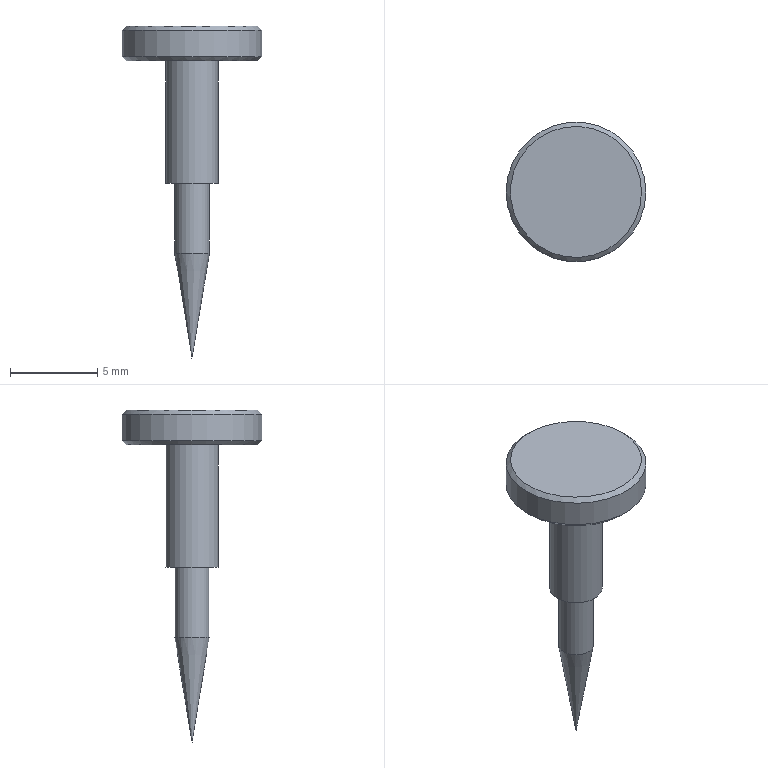Component | NX | AIR_PUMP_PART_01_20 | 1 solid | 9 faces | box 8 x 8 x 19 mm | volume 167 mm3 | cone 3 | cylinder 3 | plane 3 | commonest cylinder face diameters 2 x1 3 x1 8 x1
STEP:
#1=CARTESIAN_POINT('',(0.,0.,0.));
#2=DIRECTION('',(0.,0.,1.));
#3=DIRECTION('',(1.,0.,0.));
#4=AXIS2_PLACEMENT_3D('',#1,#2,#3);
#5=CARTESIAN_POINT('',(0.0005589,-32.2,83.052));
#6=VERTEX_POINT('',#5);
#7=CARTESIAN_POINT('',(1.001,-32.2,89.052));
#8=VERTEX_POINT('',#7);
#9=CARTESIAN_POINT('',(0.0005589,-32.2,83.052));
#10=CARTESIAN_POINT('',(1.001,-32.2,89.052));
#11=B_SPLINE_CURVE_WITH_KNOTS('',1,(#9,#10),.UNSPECIFIED.,.F.,.F.,(2,2),(-6.083,0.),.PIECEWISE_BEZIER_KNOTS.);
#12=CARTESIAN_POINT('',(0.0005589,-32.2,89.052));
#13=DIRECTION('',(0.,0.,1.));
#14=DIRECTION('',(1.,0.,0.));
#15=AXIS2_PLACEMENT_3D('',#12,#13,#14);
#16=CONICAL_SURFACE('',#15,1.,0.1651);
#17=CARTESIAN_POINT('',(6.283,0.));
#18=DIRECTION('',(0.,1.));
#19=VECTOR('',#18,1.);
#20=LINE('',#17,#19);
#21=(GEOMETRIC_REPRESENTATION_CONTEXT(2)PARAMETRIC_REPRESENTATION_CONTEXT()REPRESENTATION_CONTEXT('',''));
#22=DEFINITIONAL_REPRESENTATION('',(#20),#21);
#23=PCURVE('',#16,#22);
#24=CARTESIAN_POINT('',(0.,0.));
#25=DIRECTION('',(0.,1.));
#26=VECTOR('',#25,1.);
#27=LINE('',#24,#26);
#28=(GEOMETRIC_REPRESENTATION_CONTEXT(2)PARAMETRIC_REPRESENTATION_CONTEXT()REPRESENTATION_CONTEXT('',''));
#29=DEFINITIONAL_REPRESENTATION('',(#27),#28);
#30=PCURVE('',#16,#29);
#31=SEAM_CURVE('',#11,(#23,#30),.PCURVE_S1.);
#32=EDGE_CURVE('',#6,#8,#31,.T.);
#33=ORIENTED_EDGE('',*,*,#32,.T.);
#34=CARTESIAN_POINT('',(0.0005589,-32.2,89.052));
#35=DIRECTION('',(0.,0.,1.));
#36=DIRECTION('',(1.,0.,0.));
#37=AXIS2_PLACEMENT_3D('',#34,#35,#36);
#38=CIRCLE('',#37,1.);
#39=CARTESIAN_POINT('',(0.,0.));
#40=DIRECTION('',(1.,0.));
#41=VECTOR('',#40,1.);
#42=LINE('',#39,#41);
#43=(GEOMETRIC_REPRESENTATION_CONTEXT(2)PARAMETRIC_REPRESENTATION_CONTEXT()REPRESENTATION_CONTEXT('',''));
#44=DEFINITIONAL_REPRESENTATION('',(#42),#43);
#45=PCURVE('',#16,#44);
#46=CARTESIAN_POINT('',(0.0005589,-32.2,83.052));
#47=DIRECTION('',(0.,0.,1.));
#48=DIRECTION('',(1.,0.,0.));
#49=AXIS2_PLACEMENT_3D('',#46,#47,#48);
#50=CYLINDRICAL_SURFACE('',#49,1.);
#51=CARTESIAN_POINT('',(0.,6.));
#52=DIRECTION('',(1.,0.));
#53=VECTOR('',#52,1.);
#54=LINE('',#51,#53);
#55=(GEOMETRIC_REPRESENTATION_CONTEXT(2)PARAMETRIC_REPRESENTATION_CONTEXT()REPRESENTATION_CONTEXT('',''));
#56=DEFINITIONAL_REPRESENTATION('',(#54),#55);
#57=PCURVE('',#50,#56);
#58=SURFACE_CURVE('',#38,(#45,#57),.PCURVE_S1.);
#59=EDGE_CURVE('',#8,#8,#58,.T.);
#60=ORIENTED_EDGE('',*,*,#59,.F.);
#61=ORIENTED_EDGE('',*,*,#32,.F.);
#62=EDGE_LOOP('',(#33,#60,#61));
#63=FACE_BOUND('',#62,.T.);
#64=ADVANCED_FACE('',(#63),#16,.T.);
#65=ORIENTED_EDGE('',*,*,#59,.T.);
#66=CARTESIAN_POINT('',(1.001,-32.2,93.052));
#67=VERTEX_POINT('',#66);
#68=CARTESIAN_POINT('',(1.001,-32.2,89.052));
#69=CARTESIAN_POINT('',(1.001,-32.2,93.052));
#70=B_SPLINE_CURVE_WITH_KNOTS('',1,(#68,#69),.UNSPECIFIED.,.F.,.F.,(2,2),(6.,10.),.PIECEWISE_BEZIER_KNOTS.);
#71=CARTESIAN_POINT('',(6.283,0.));
#72=DIRECTION('',(0.,1.));
#73=VECTOR('',#72,1.);
#74=LINE('',#71,#73);
#75=(GEOMETRIC_REPRESENTATION_CONTEXT(2)PARAMETRIC_REPRESENTATION_CONTEXT()REPRESENTATION_CONTEXT('',''));
#76=DEFINITIONAL_REPRESENTATION('',(#74),#75);
#77=PCURVE('',#50,#76);
#78=CARTESIAN_POINT('',(0.,0.));
#79=DIRECTION('',(0.,1.));
#80=VECTOR('',#79,1.);
#81=LINE('',#78,#80);
#82=(GEOMETRIC_REPRESENTATION_CONTEXT(2)PARAMETRIC_REPRESENTATION_CONTEXT()REPRESENTATION_CONTEXT('',''));
#83=DEFINITIONAL_REPRESENTATION('',(#81),#82);
#84=PCURVE('',#50,#83);
#85=SEAM_CURVE('',#70,(#77,#84),.PCURVE_S1.);
#86=EDGE_CURVE('',#8,#67,#85,.T.);
#87=ORIENTED_EDGE('',*,*,#86,.T.);
#88=CARTESIAN_POINT('',(0.0005589,-32.2,93.052));
#89=DIRECTION('',(0.,0.,1.));
#90=DIRECTION('',(1.,0.,0.));
#91=AXIS2_PLACEMENT_3D('',#88,#89,#90);
#92=CIRCLE('',#91,1.);
#93=CARTESIAN_POINT('',(0.,10.));
#94=DIRECTION('',(1.,0.));
#95=VECTOR('',#94,1.);
#96=LINE('',#93,#95);
#97=(GEOMETRIC_REPRESENTATION_CONTEXT(2)PARAMETRIC_REPRESENTATION_CONTEXT()REPRESENTATION_CONTEXT('',''));
#98=DEFINITIONAL_REPRESENTATION('',(#96),#97);
#99=PCURVE('',#50,#98);
#100=CARTESIAN_POINT('',(0.0005589,-33.7,93.052));
#101=DIRECTION('',(0.,0.,-1.));
#102=DIRECTION('',(-1.,0.,0.));
#103=AXIS2_PLACEMENT_3D('',#100,#101,#102);
#104=PLANE('',#103);
#105=CARTESIAN_POINT('',(-1.,1.5));
#106=CARTESIAN_POINT('',(-1.,3.232));
#107=CARTESIAN_POINT('',(0.5,2.366));
#108=CARTESIAN_POINT('',(2.,1.5));
#109=CARTESIAN_POINT('',(0.5,0.634));
#110=CARTESIAN_POINT('',(-1.,-0.2321));
#111=CARTESIAN_POINT('',(-1.,1.5));
#112=(BOUNDED_CURVE()B_SPLINE_CURVE(2,(#105,#106,#107,#108,#109,#110,#111),.UNSPECIFIED.,.T.,.F.)B_SPLINE_CURVE_WITH_KNOTS((1,2,2,2,2,1),(-2.094,0.,2.094,4.189,6.283,8.378),.UNSPECIFIED.)CURVE()GEOMETRIC_REPRESENTATION_ITEM()RATIONAL_B_SPLINE_CURVE((1.,0.5,1.,0.5,1.,0.5,1.))REPRESENTATION_ITEM(''));
#113=(GEOMETRIC_REPRESENTATION_CONTEXT(2)PARAMETRIC_REPRESENTATION_CONTEXT()REPRESENTATION_CONTEXT('',''));
#114=DEFINITIONAL_REPRESENTATION('',(#112),#113);
#115=PCURVE('',#104,#114);
#116=SURFACE_CURVE('',#92,(#99,#115),.PCURVE_S1.);
#117=EDGE_CURVE('',#67,#67,#116,.T.);
#118=ORIENTED_EDGE('',*,*,#117,.F.);
#119=ORIENTED_EDGE('',*,*,#86,.F.);
#120=EDGE_LOOP('',(#65,#87,#118,#119));
#121=FACE_BOUND('',#120,.T.);
#122=ADVANCED_FACE('',(#121),#50,.T.);
#123=ORIENTED_EDGE('',*,*,#117,.T.);
#124=EDGE_LOOP('',(#123));
#125=FACE_BOUND('',#124,.T.);
#126=CARTESIAN_POINT('',(1.501,-32.2,93.052));
#127=VERTEX_POINT('',#126);
#128=CARTESIAN_POINT('',(0.0005589,-32.2,93.052));
#129=DIRECTION('',(0.,0.,1.));
#130=DIRECTION('',(1.,0.,0.));
#131=AXIS2_PLACEMENT_3D('',#128,#129,#130);
#132=CIRCLE('',#131,1.5);
#133=CARTESIAN_POINT('',(-1.5,1.5));
#134=CARTESIAN_POINT('',(-1.5,4.098));
#135=CARTESIAN_POINT('',(0.75,2.799));
#136=CARTESIAN_POINT('',(3.,1.5));
#137=CARTESIAN_POINT('',(0.75,0.201));
#138=CARTESIAN_POINT('',(-1.5,-1.098));
#139=CARTESIAN_POINT('',(-1.5,1.5));
#140=(BOUNDED_CURVE()B_SPLINE_CURVE(2,(#133,#134,#135,#136,#137,#138,#139),.UNSPECIFIED.,.T.,.F.)B_SPLINE_CURVE_WITH_KNOTS((1,2,2,2,2,1),(-2.094,0.,2.094,4.189,6.283,8.378),.UNSPECIFIED.)CURVE()GEOMETRIC_REPRESENTATION_ITEM()RATIONAL_B_SPLINE_CURVE((1.,0.5,1.,0.5,1.,0.5,1.))REPRESENTATION_ITEM(''));
#141=(GEOMETRIC_REPRESENTATION_CONTEXT(2)PARAMETRIC_REPRESENTATION_CONTEXT()REPRESENTATION_CONTEXT('',''));
#142=DEFINITIONAL_REPRESENTATION('',(#140),#141);
#143=PCURVE('',#104,#142);
#144=CARTESIAN_POINT('',(0.0005589,-32.2,83.052));
#145=DIRECTION('',(0.,0.,1.));
#146=DIRECTION('',(1.,0.,0.));
#147=AXIS2_PLACEMENT_3D('',#144,#145,#146);
#148=CYLINDRICAL_SURFACE('',#147,1.5);
#149=CARTESIAN_POINT('',(0.,10.));
#150=DIRECTION('',(1.,0.));
#151=VECTOR('',#150,1.);
#152=LINE('',#149,#151);
#153=(GEOMETRIC_REPRESENTATION_CONTEXT(2)PARAMETRIC_REPRESENTATION_CONTEXT()REPRESENTATION_CONTEXT('',''));
#154=DEFINITIONAL_REPRESENTATION('',(#152),#153);
#155=PCURVE('',#148,#154);
#156=SURFACE_CURVE('',#132,(#143,#155),.PCURVE_S1.);
#157=EDGE_CURVE('',#127,#127,#156,.T.);
#158=ORIENTED_EDGE('',*,*,#157,.F.);
#159=EDGE_LOOP('',(#158));
#160=FACE_BOUND('',#159,.T.);
#161=ADVANCED_FACE('',(#125,#160),#104,.T.);
#162=ORIENTED_EDGE('',*,*,#157,.T.);
#163=CARTESIAN_POINT('',(1.501,-32.2,100.052));
#164=VERTEX_POINT('',#163);
#165=CARTESIAN_POINT('',(1.501,-32.2,93.052));
#166=CARTESIAN_POINT('',(1.501,-32.2,100.052));
#167=B_SPLINE_CURVE_WITH_KNOTS('',1,(#165,#166),.UNSPECIFIED.,.F.,.F.,(2,2),(10.,17.),.PIECEWISE_BEZIER_KNOTS.);
#168=CARTESIAN_POINT('',(6.283,0.));
#169=DIRECTION('',(0.,1.));
#170=VECTOR('',#169,1.);
#171=LINE('',#168,#170);
#172=(GEOMETRIC_REPRESENTATION_CONTEXT(2)PARAMETRIC_REPRESENTATION_CONTEXT()REPRESENTATION_CONTEXT('',''));
#173=DEFINITIONAL_REPRESENTATION('',(#171),#172);
#174=PCURVE('',#148,#173);
#175=CARTESIAN_POINT('',(0.,0.));
#176=DIRECTION('',(0.,1.));
#177=VECTOR('',#176,1.);
#178=LINE('',#175,#177);
#179=(GEOMETRIC_REPRESENTATION_CONTEXT(2)PARAMETRIC_REPRESENTATION_CONTEXT()REPRESENTATION_CONTEXT('',''));
#180=DEFINITIONAL_REPRESENTATION('',(#178),#179);
#181=PCURVE('',#148,#180);
#182=SEAM_CURVE('',#167,(#174,#181),.PCURVE_S1.);
#183=EDGE_CURVE('',#127,#164,#182,.T.);
#184=ORIENTED_EDGE('',*,*,#183,.T.);
#185=CARTESIAN_POINT('',(0.0005589,-32.2,100.052));
#186=DIRECTION('',(0.,0.,1.));
#187=DIRECTION('',(1.,0.,0.));
#188=AXIS2_PLACEMENT_3D('',#185,#186,#187);
#189=CIRCLE('',#188,1.5);
#190=CARTESIAN_POINT('',(0.,17.));
#191=DIRECTION('',(1.,0.));
#192=VECTOR('',#191,1.);
#193=LINE('',#190,#192);
#194=(GEOMETRIC_REPRESENTATION_CONTEXT(2)PARAMETRIC_REPRESENTATION_CONTEXT()REPRESENTATION_CONTEXT('',''));
#195=DEFINITIONAL_REPRESENTATION('',(#193),#194);
#196=PCURVE('',#148,#195);
#197=CARTESIAN_POINT('',(0.0005589,-36.2,100.052));
#198=DIRECTION('',(0.,0.,-1.));
#199=DIRECTION('',(-1.,0.,0.));
#200=AXIS2_PLACEMENT_3D('',#197,#198,#199);
#201=PLANE('',#200);
#202=CARTESIAN_POINT('',(-1.5,4.));
#203=CARTESIAN_POINT('',(-1.5,6.598));
#204=CARTESIAN_POINT('',(0.75,5.299));
#205=CARTESIAN_POINT('',(3.,4.));
#206=CARTESIAN_POINT('',(0.75,2.701));
#207=CARTESIAN_POINT('',(-1.5,1.402));
#208=CARTESIAN_POINT('',(-1.5,4.));
#209=(BOUNDED_CURVE()B_SPLINE_CURVE(2,(#202,#203,#204,#205,#206,#207,#208),.UNSPECIFIED.,.T.,.F.)B_SPLINE_CURVE_WITH_KNOTS((1,2,2,2,2,1),(-2.094,0.,2.094,4.189,6.283,8.378),.UNSPECIFIED.)CURVE()GEOMETRIC_REPRESENTATION_ITEM()RATIONAL_B_SPLINE_CURVE((1.,0.5,1.,0.5,1.,0.5,1.))REPRESENTATION_ITEM(''));
#210=(GEOMETRIC_REPRESENTATION_CONTEXT(2)PARAMETRIC_REPRESENTATION_CONTEXT()REPRESENTATION_CONTEXT('',''));
#211=DEFINITIONAL_REPRESENTATION('',(#209),#210);
#212=PCURVE('',#201,#211);
#213=SURFACE_CURVE('',#189,(#196,#212),.PCURVE_S1.);
#214=EDGE_CURVE('',#164,#164,#213,.T.);
#215=ORIENTED_EDGE('',*,*,#214,.F.);
#216=ORIENTED_EDGE('',*,*,#183,.F.);
#217=EDGE_LOOP('',(#162,#184,#215,#216));
#218=FACE_BOUND('',#217,.T.);
#219=ADVANCED_FACE('',(#218),#148,.T.);
#220=CARTESIAN_POINT('',(-3.749,-32.2,100.052));
#221=VERTEX_POINT('',#220);
#222=CARTESIAN_POINT('',(0.0005589,-32.2,100.052));
#223=DIRECTION('',(0.,0.,-1.));
#224=DIRECTION('',(-1.,0.,0.));
#225=AXIS2_PLACEMENT_3D('',#222,#223,#224);
#226=CIRCLE('',#225,3.75);
#227=CARTESIAN_POINT('',(0.,4.));
#228=DIRECTION('',(1.,0.));
#229=AXIS2_PLACEMENT_2D('',#227,#228);
#230=CIRCLE('',#229,3.75);
#231=(GEOMETRIC_REPRESENTATION_CONTEXT(2)PARAMETRIC_REPRESENTATION_CONTEXT()REPRESENTATION_CONTEXT('',''));
#232=DEFINITIONAL_REPRESENTATION('',(#230),#231);
#233=PCURVE('',#201,#232);
#234=CARTESIAN_POINT('',(0.0005589,-32.2,100.302));
#235=DIRECTION('',(0.,0.,1.));
#236=DIRECTION('',(1.,0.,0.));
#237=AXIS2_PLACEMENT_3D('',#234,#235,#236);
#238=CONICAL_SURFACE('',#237,4.,0.7854);
#239=CARTESIAN_POINT('',(9.425,-0.25));
#240=DIRECTION('',(-1.,0.));
#241=VECTOR('',#240,1.);
#242=LINE('',#239,#241);
#243=(GEOMETRIC_REPRESENTATION_CONTEXT(2)PARAMETRIC_REPRESENTATION_CONTEXT()REPRESENTATION_CONTEXT('',''));
#244=DEFINITIONAL_REPRESENTATION('',(#242),#243);
#245=PCURVE('',#238,#244);
#246=SURFACE_CURVE('',#226,(#233,#245),.PCURVE_S1.);
#247=EDGE_CURVE('',#221,#221,#246,.T.);
#248=ORIENTED_EDGE('',*,*,#247,.T.);
#249=EDGE_LOOP('',(#248));
#250=FACE_BOUND('',#249,.T.);
#251=ORIENTED_EDGE('',*,*,#214,.T.);
#252=EDGE_LOOP('',(#251));
#253=FACE_BOUND('',#252,.T.);
#254=ADVANCED_FACE('',(#250,#253),#201,.T.);
#255=CARTESIAN_POINT('',(4.001,-32.2,101.802));
#256=VERTEX_POINT('',#255);
#257=CARTESIAN_POINT('',(0.0005589,-32.2,101.802));
#258=DIRECTION('',(0.,0.,-1.));
#259=DIRECTION('',(1.,0.,0.));
#260=AXIS2_PLACEMENT_3D('',#257,#258,#259);
#261=CIRCLE('',#260,4.);
#262=CARTESIAN_POINT('',(0.0005589,-32.2,83.052));
#263=DIRECTION('',(0.,0.,1.));
#264=DIRECTION('',(1.,0.,0.));
#265=AXIS2_PLACEMENT_3D('',#262,#263,#264);
#266=CYLINDRICAL_SURFACE('',#265,4.);
#267=CARTESIAN_POINT('',(6.283,18.75));
#268=DIRECTION('',(-1.,0.));
#269=VECTOR('',#268,1.);
#270=LINE('',#267,#269);
#271=(GEOMETRIC_REPRESENTATION_CONTEXT(2)PARAMETRIC_REPRESENTATION_CONTEXT()REPRESENTATION_CONTEXT('',''));
#272=DEFINITIONAL_REPRESENTATION('',(#270),#271);
#273=PCURVE('',#266,#272);
#274=CARTESIAN_POINT('',(0.0005589,-32.2,102.052));
#275=DIRECTION('',(0.,0.,-1.));
#276=DIRECTION('',(-1.,0.,0.));
#277=AXIS2_PLACEMENT_3D('',#274,#275,#276);
#278=CONICAL_SURFACE('',#277,3.75,0.7854);
#279=CARTESIAN_POINT('',(3.142,0.25));
#280=DIRECTION('',(1.,0.));
#281=VECTOR('',#280,1.);
#282=LINE('',#279,#281);
#283=(GEOMETRIC_REPRESENTATION_CONTEXT(2)PARAMETRIC_REPRESENTATION_CONTEXT()REPRESENTATION_CONTEXT('',''));
#284=DEFINITIONAL_REPRESENTATION('',(#282),#283);
#285=PCURVE('',#278,#284);
#286=SURFACE_CURVE('',#261,(#273,#285),.PCURVE_S1.);
#287=EDGE_CURVE('',#256,#256,#286,.T.);
#288=ORIENTED_EDGE('',*,*,#287,.T.);
#289=CARTESIAN_POINT('',(4.001,-32.2,100.302));
#290=VERTEX_POINT('',#289);
#291=CARTESIAN_POINT('',(4.001,-32.2,100.302));
#292=CARTESIAN_POINT('',(4.001,-32.2,101.802));
#293=B_SPLINE_CURVE_WITH_KNOTS('',1,(#291,#292),.UNSPECIFIED.,.F.,.F.,(2,2),(17.25,18.75),.PIECEWISE_BEZIER_KNOTS.);
#294=CARTESIAN_POINT('',(0.,0.));
#295=DIRECTION('',(0.,1.));
#296=VECTOR('',#295,1.);
#297=LINE('',#294,#296);
#298=(GEOMETRIC_REPRESENTATION_CONTEXT(2)PARAMETRIC_REPRESENTATION_CONTEXT()REPRESENTATION_CONTEXT('',''));
#299=DEFINITIONAL_REPRESENTATION('',(#297),#298);
#300=PCURVE('',#266,#299);
#301=CARTESIAN_POINT('',(6.283,0.));
#302=DIRECTION('',(0.,1.));
#303=VECTOR('',#302,1.);
#304=LINE('',#301,#303);
#305=(GEOMETRIC_REPRESENTATION_CONTEXT(2)PARAMETRIC_REPRESENTATION_CONTEXT()REPRESENTATION_CONTEXT('',''));
#306=DEFINITIONAL_REPRESENTATION('',(#304),#305);
#307=PCURVE('',#266,#306);
#308=SEAM_CURVE('',#293,(#300,#307),.PCURVE_S1.);
#309=EDGE_CURVE('',#290,#256,#308,.T.);
#310=ORIENTED_EDGE('',*,*,#309,.F.);
#311=CARTESIAN_POINT('',(-3.999,-32.2,100.302));
#312=VERTEX_POINT('',#311);
#313=CARTESIAN_POINT('',(0.0005589,-32.2,100.302));
#314=DIRECTION('',(0.,0.,1.));
#315=DIRECTION('',(-1.,0.,0.));
#316=AXIS2_PLACEMENT_3D('',#313,#314,#315);
#317=CIRCLE('',#316,4.);
#318=CARTESIAN_POINT('',(-3.142,17.25));
#319=DIRECTION('',(1.,0.));
#320=VECTOR('',#319,1.);
#321=LINE('',#318,#320);
#322=(GEOMETRIC_REPRESENTATION_CONTEXT(2)PARAMETRIC_REPRESENTATION_CONTEXT()REPRESENTATION_CONTEXT('',''));
#323=DEFINITIONAL_REPRESENTATION('',(#321),#322);
#324=PCURVE('',#266,#323);
#325=CARTESIAN_POINT('',(3.142,-0.));
#326=DIRECTION('',(1.,0.));
#327=VECTOR('',#326,1.);
#328=LINE('',#325,#327);
#329=(GEOMETRIC_REPRESENTATION_CONTEXT(2)PARAMETRIC_REPRESENTATION_CONTEXT()REPRESENTATION_CONTEXT('',''));
#330=DEFINITIONAL_REPRESENTATION('',(#328),#329);
#331=PCURVE('',#238,#330);
#332=SURFACE_CURVE('',#317,(#324,#331),.PCURVE_S1.);
#333=EDGE_CURVE('',#290,#312,#332,.T.);
#334=ORIENTED_EDGE('',*,*,#333,.T.);
#335=CARTESIAN_POINT('',(0.0005589,-32.2,100.302));
#336=DIRECTION('',(0.,0.,1.));
#337=DIRECTION('',(-1.,0.,0.));
#338=AXIS2_PLACEMENT_3D('',#335,#336,#337);
#339=CIRCLE('',#338,4.);
#340=CARTESIAN_POINT('',(3.142,17.25));
#341=DIRECTION('',(1.,0.));
#342=VECTOR('',#341,1.);
#343=LINE('',#340,#342);
#344=(GEOMETRIC_REPRESENTATION_CONTEXT(2)PARAMETRIC_REPRESENTATION_CONTEXT()REPRESENTATION_CONTEXT('',''));
#345=DEFINITIONAL_REPRESENTATION('',(#343),#344);
#346=PCURVE('',#266,#345);
#347=CARTESIAN_POINT('',(3.142,0.));
#348=DIRECTION('',(1.,-0.));
#349=VECTOR('',#348,1.);
#350=LINE('',#347,#349);
#351=(GEOMETRIC_REPRESENTATION_CONTEXT(2)PARAMETRIC_REPRESENTATION_CONTEXT()REPRESENTATION_CONTEXT('',''));
#352=DEFINITIONAL_REPRESENTATION('',(#350),#351);
#353=PCURVE('',#238,#352);
#354=SURFACE_CURVE('',#339,(#346,#353),.PCURVE_S1.);
#355=EDGE_CURVE('',#312,#290,#354,.T.);
#356=ORIENTED_EDGE('',*,*,#355,.T.);
#357=ORIENTED_EDGE('',*,*,#309,.T.);
#358=EDGE_LOOP('',(#288,#310,#334,#356,#357));
#359=FACE_BOUND('',#358,.T.);
#360=ADVANCED_FACE('',(#359),#266,.T.);
#361=CARTESIAN_POINT('',(3.751,-32.2,102.052));
#362=VERTEX_POINT('',#361);
#363=CARTESIAN_POINT('',(0.0005589,-32.2,102.052));
#364=DIRECTION('',(0.,0.,1.));
#365=DIRECTION('',(1.,0.,0.));
#366=AXIS2_PLACEMENT_3D('',#363,#364,#365);
#367=CIRCLE('',#366,3.75);
#368=CARTESIAN_POINT('',(0.0005589,-32.2,102.052));
#369=DIRECTION('',(0.,0.,1.));
#370=DIRECTION('',(1.,0.,0.));
#371=AXIS2_PLACEMENT_3D('',#368,#369,#370);
#372=PLANE('',#371);
#373=CARTESIAN_POINT('',(0.,0.));
#374=DIRECTION('',(1.,0.));
#375=AXIS2_PLACEMENT_2D('',#373,#374);
#376=CIRCLE('',#375,3.75);
#377=(GEOMETRIC_REPRESENTATION_CONTEXT(2)PARAMETRIC_REPRESENTATION_CONTEXT()REPRESENTATION_CONTEXT('',''));
#378=DEFINITIONAL_REPRESENTATION('',(#376),#377);
#379=PCURVE('',#372,#378);
#380=CARTESIAN_POINT('',(9.425,0.));
#381=DIRECTION('',(-1.,0.));
#382=VECTOR('',#381,1.);
#383=LINE('',#380,#382);
#384=(GEOMETRIC_REPRESENTATION_CONTEXT(2)PARAMETRIC_REPRESENTATION_CONTEXT()REPRESENTATION_CONTEXT('',''));
#385=DEFINITIONAL_REPRESENTATION('',(#383),#384);
#386=PCURVE('',#278,#385);
#387=SURFACE_CURVE('',#367,(#379,#386),.PCURVE_S1.);
#388=EDGE_CURVE('',#362,#362,#387,.T.);
#389=ORIENTED_EDGE('',*,*,#388,.T.);
#390=EDGE_LOOP('',(#389));
#391=FACE_BOUND('',#390,.T.);
#392=ADVANCED_FACE('',(#391),#372,.T.);
#393=ORIENTED_EDGE('',*,*,#287,.F.);
#394=CARTESIAN_POINT('',(3.751,-32.2,102.052));
#395=CARTESIAN_POINT('',(4.001,-32.2,101.802));
#396=B_SPLINE_CURVE_WITH_KNOTS('',1,(#394,#395),.UNSPECIFIED.,.F.,.F.,(2,2),(0.,0.3536),.PIECEWISE_BEZIER_KNOTS.);
#397=CARTESIAN_POINT('',(3.142,0.));
#398=DIRECTION('',(0.,1.));
#399=VECTOR('',#398,1.);
#400=LINE('',#397,#399);
#401=(GEOMETRIC_REPRESENTATION_CONTEXT(2)PARAMETRIC_REPRESENTATION_CONTEXT()REPRESENTATION_CONTEXT('',''));
#402=DEFINITIONAL_REPRESENTATION('',(#400),#401);
#403=PCURVE('',#278,#402);
#404=CARTESIAN_POINT('',(9.425,0.));
#405=DIRECTION('',(0.,1.));
#406=VECTOR('',#405,1.);
#407=LINE('',#404,#406);
#408=(GEOMETRIC_REPRESENTATION_CONTEXT(2)PARAMETRIC_REPRESENTATION_CONTEXT()REPRESENTATION_CONTEXT('',''));
#409=DEFINITIONAL_REPRESENTATION('',(#407),#408);
#410=PCURVE('',#278,#409);
#411=SEAM_CURVE('',#396,(#403,#410),.PCURVE_S1.);
#412=EDGE_CURVE('',#362,#256,#411,.T.);
#413=ORIENTED_EDGE('',*,*,#412,.F.);
#414=ORIENTED_EDGE('',*,*,#388,.F.);
#415=ORIENTED_EDGE('',*,*,#412,.T.);
#416=EDGE_LOOP('',(#393,#413,#414,#415));
#417=FACE_BOUND('',#416,.T.);
#418=ADVANCED_FACE('',(#417),#278,.T.);
#419=ORIENTED_EDGE('',*,*,#247,.F.);
#420=CARTESIAN_POINT('',(-3.749,-32.2,100.052));
#421=CARTESIAN_POINT('',(-3.999,-32.2,100.302));
#422=B_SPLINE_CURVE_WITH_KNOTS('',1,(#420,#421),.UNSPECIFIED.,.F.,.F.,(2,2),(-0.3536,0.),.PIECEWISE_BEZIER_KNOTS.);
#423=CARTESIAN_POINT('',(9.425,0.));
#424=DIRECTION('',(0.,1.));
#425=VECTOR('',#424,1.);
#426=LINE('',#423,#425);
#427=(GEOMETRIC_REPRESENTATION_CONTEXT(2)PARAMETRIC_REPRESENTATION_CONTEXT()REPRESENTATION_CONTEXT('',''));
#428=DEFINITIONAL_REPRESENTATION('',(#426),#427);
#429=PCURVE('',#238,#428);
#430=CARTESIAN_POINT('',(3.142,0.));
#431=DIRECTION('',(0.,1.));
#432=VECTOR('',#431,1.);
#433=LINE('',#430,#432);
#434=(GEOMETRIC_REPRESENTATION_CONTEXT(2)PARAMETRIC_REPRESENTATION_CONTEXT()REPRESENTATION_CONTEXT('',''));
#435=DEFINITIONAL_REPRESENTATION('',(#433),#434);
#436=PCURVE('',#238,#435);
#437=SEAM_CURVE('',#422,(#429,#436),.PCURVE_S1.);
#438=EDGE_CURVE('',#221,#312,#437,.T.);
#439=ORIENTED_EDGE('',*,*,#438,.T.);
#440=ORIENTED_EDGE('',*,*,#333,.F.);
#441=ORIENTED_EDGE('',*,*,#355,.F.);
#442=ORIENTED_EDGE('',*,*,#438,.F.);
#443=EDGE_LOOP('',(#419,#439,#440,#441,#442));
#444=FACE_BOUND('',#443,.T.);
#445=ADVANCED_FACE('',(#444),#238,.T.);
#446=CLOSED_SHELL('',(#64,#122,#161,#219,#254,#360,#392,#418,#445));
#447=MANIFOLD_SOLID_BREP('',#446);
#448=(LENGTH_UNIT()NAMED_UNIT(*)SI_UNIT(.MILLI.,.METRE.));
#449=UNCERTAINTY_MEASURE_WITH_UNIT(LENGTH_MEASURE(0.00001),#448,'','');
#450=(NAMED_UNIT(*)PLANE_ANGLE_UNIT()SI_UNIT($,.RADIAN.));
#451=(NAMED_UNIT(*)SI_UNIT($,.STERADIAN.)SOLID_ANGLE_UNIT());
#452=(GEOMETRIC_REPRESENTATION_CONTEXT(3)GLOBAL_UNCERTAINTY_ASSIGNED_CONTEXT((#449))GLOBAL_UNIT_ASSIGNED_CONTEXT((#448,#450,#451))REPRESENTATION_CONTEXT('',''));
#453=ADVANCED_BREP_SHAPE_REPRESENTATION('',(#4,#447),#452);